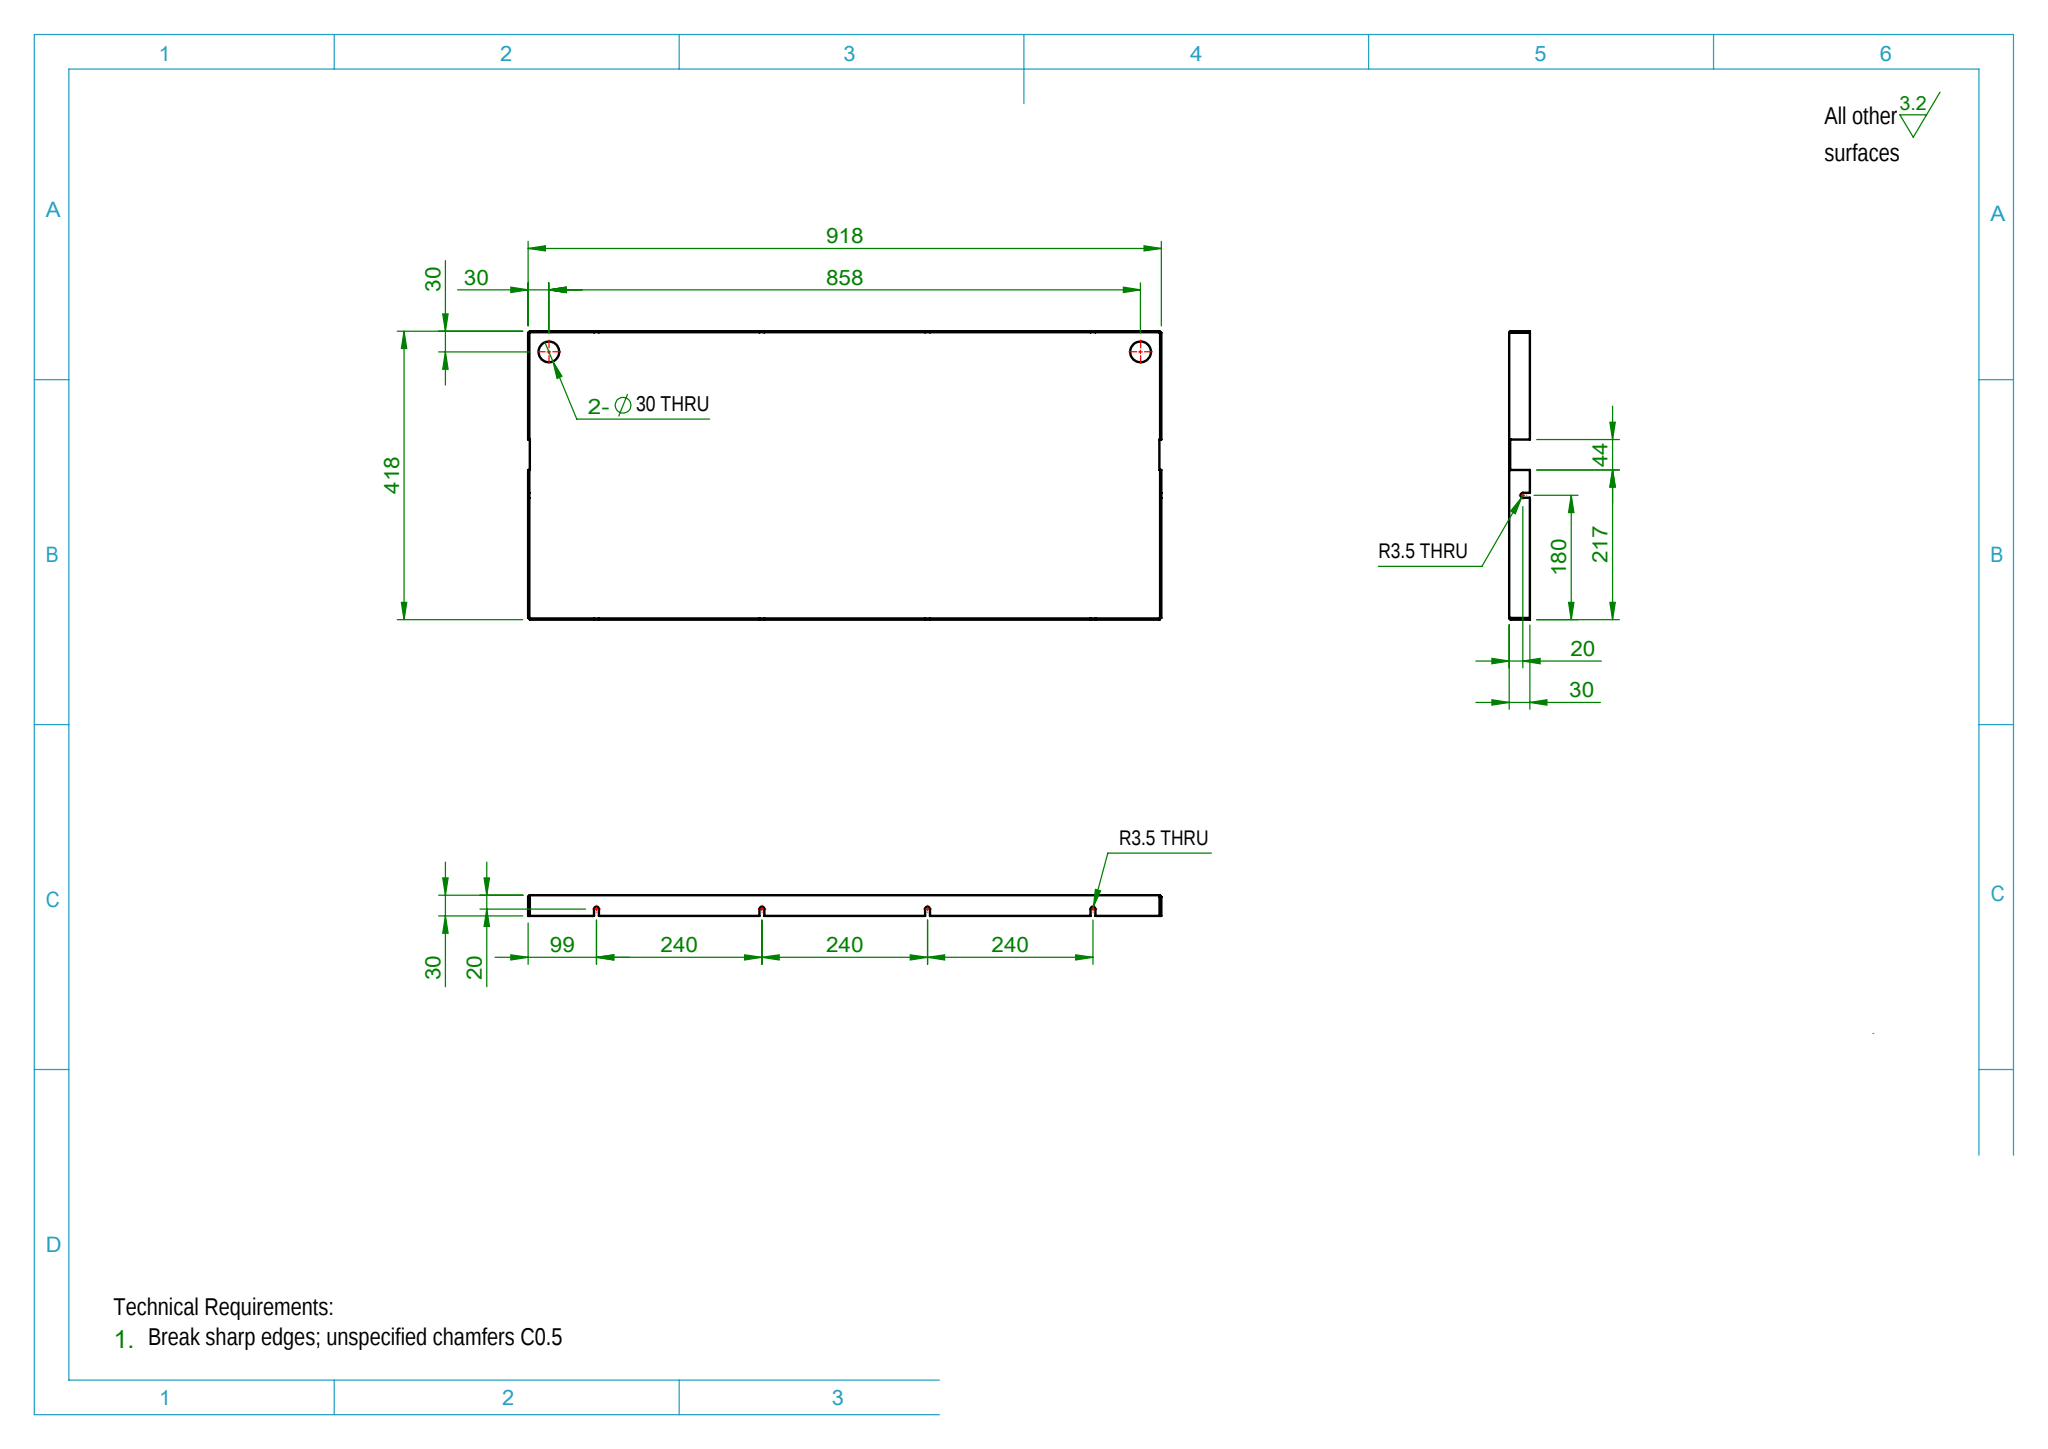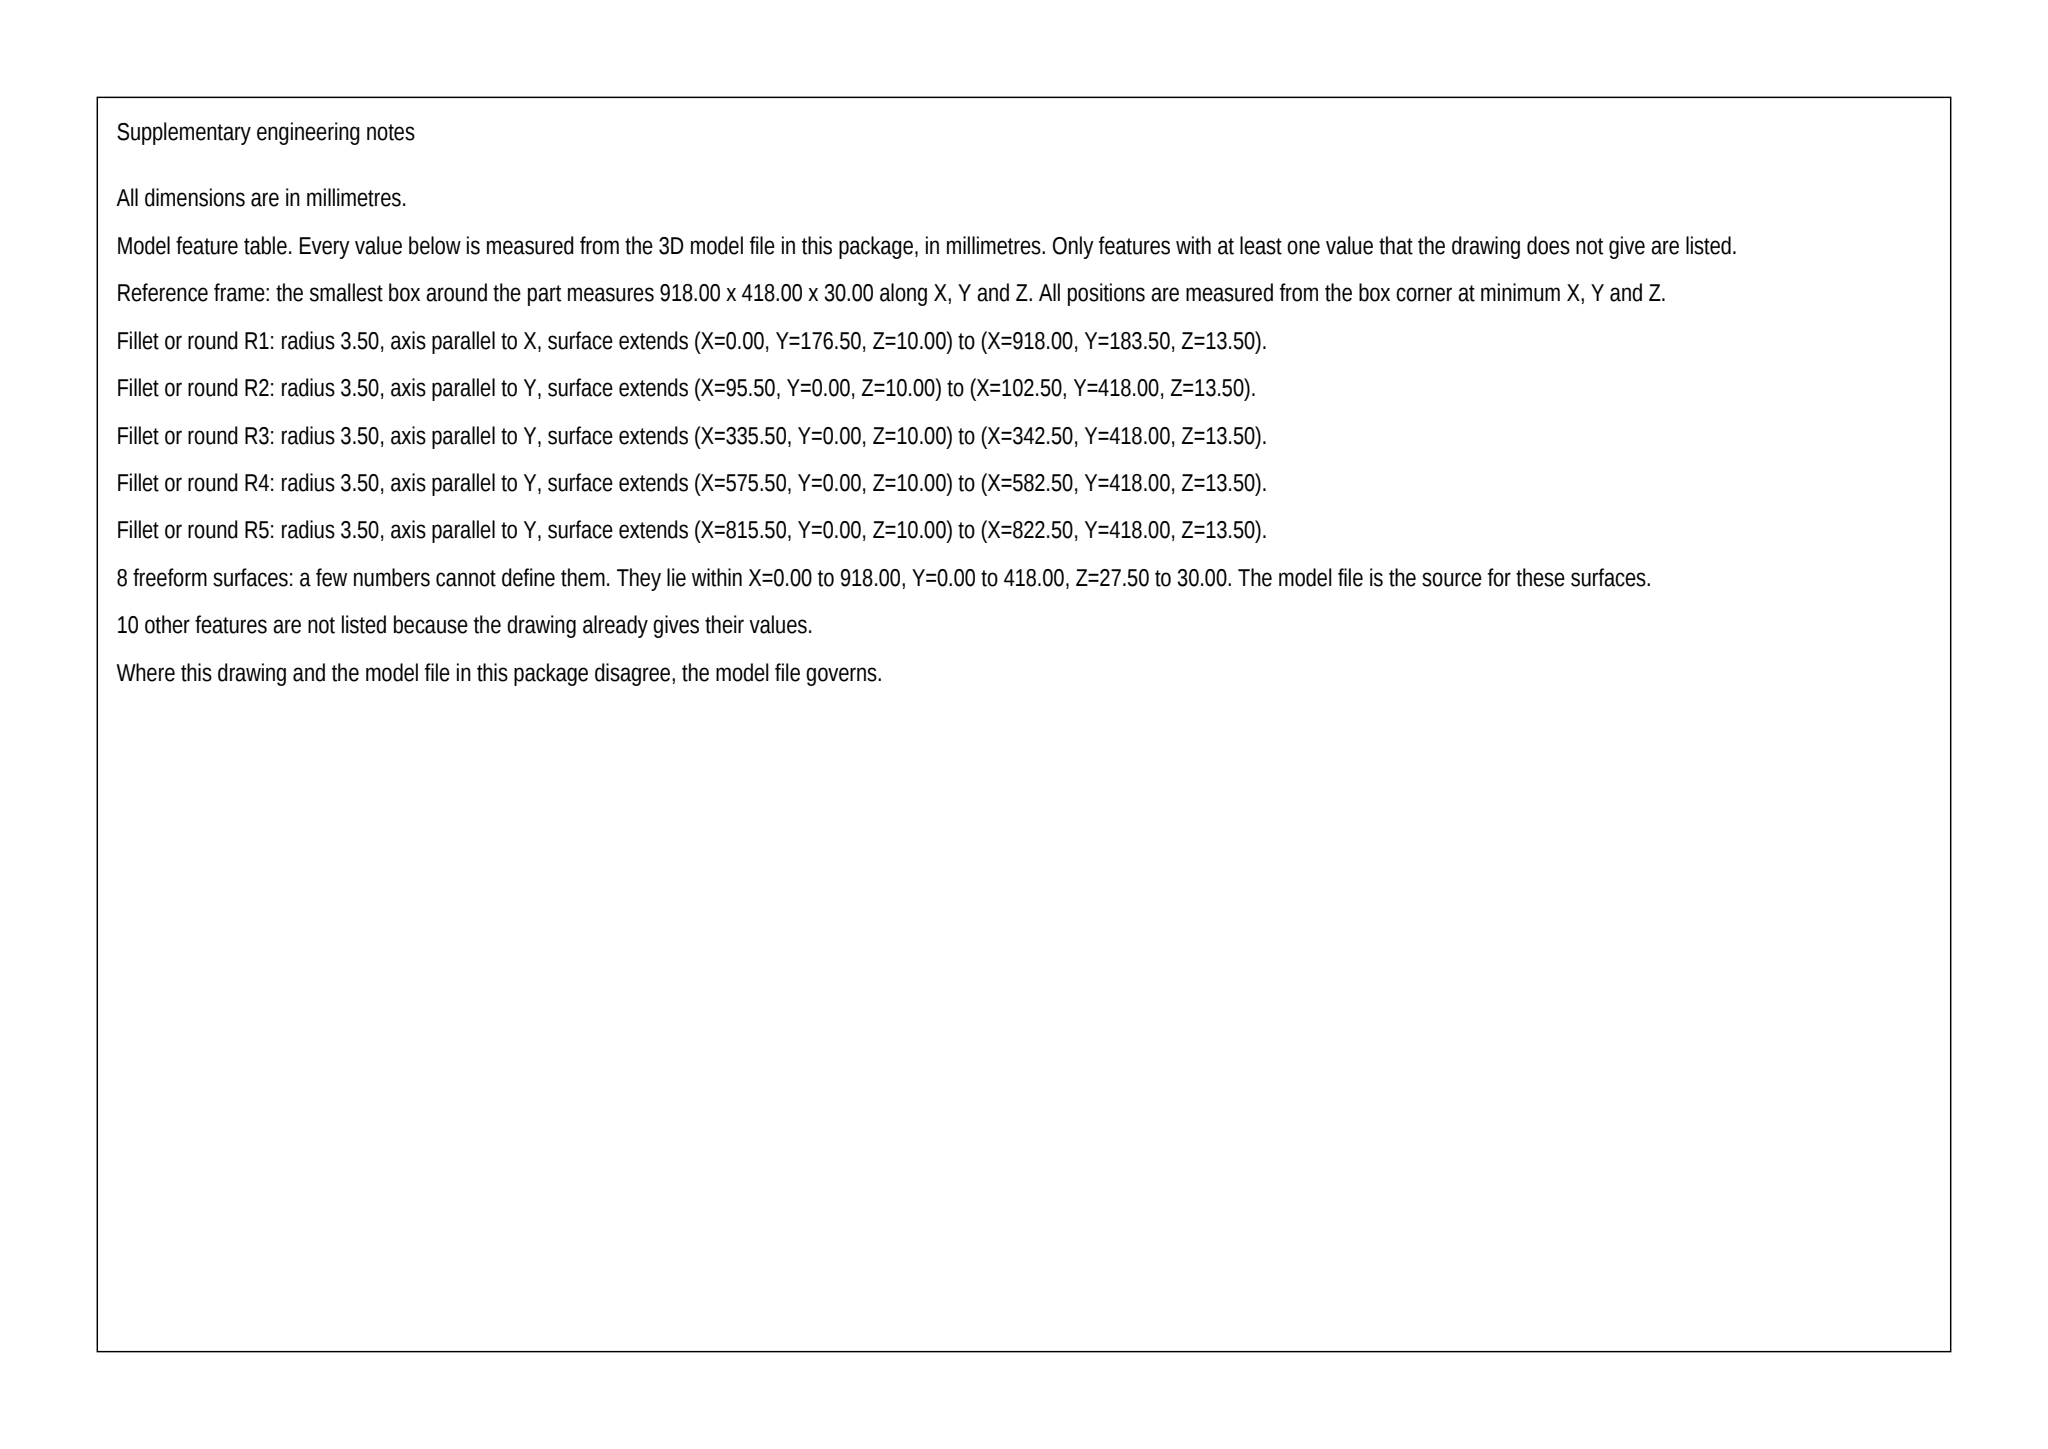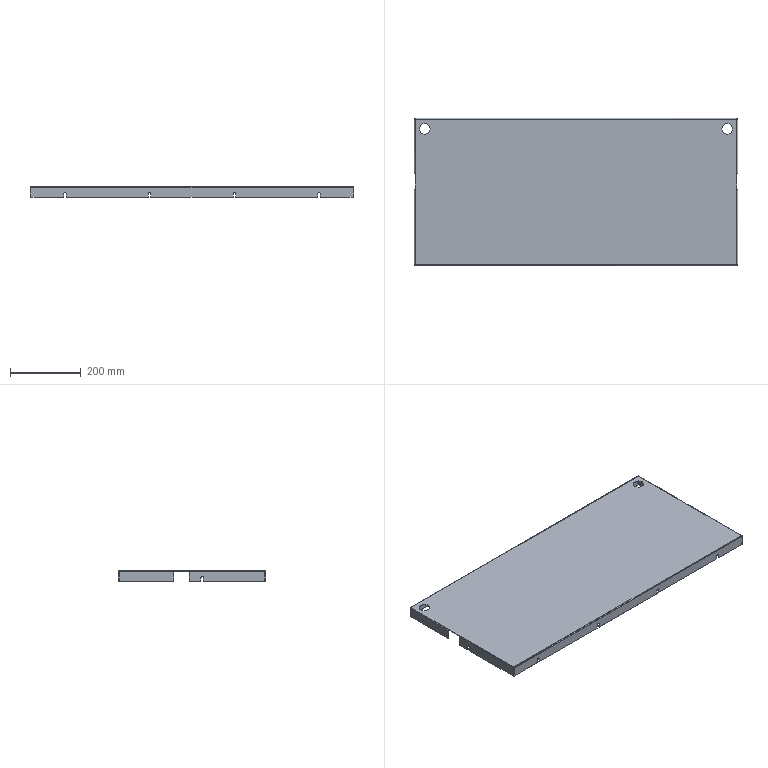Part | SolidWorks | mm | 1 solid | 104 faces | box 918 x 418 x 30 mm | volume 678583 mm3 | plane 68 | cylinder 28 | spline 8 | commonest cylinder face diameters 7 x12 5 x6 2 x6 30 x4